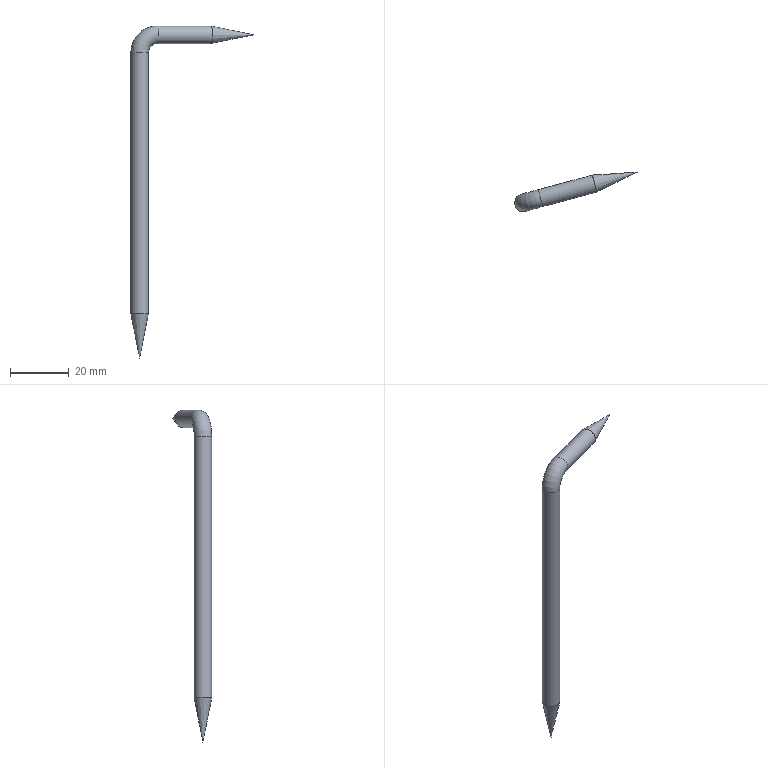Component | NX | 3 | 3 solids | 9 faces | box 41.64 x 13.41 x 113 mm | volume 3603 mm3 | plane 4 | cone 2 | cylinder 2 | torus 1 | commonest cylinder face diameters 6 x2
STEP:
#1=CARTESIAN_POINT('',(0.,0.,0.));
#2=DIRECTION('',(0.,0.,1.));
#3=DIRECTION('',(1.,0.,0.));
#4=AXIS2_PLACEMENT_3D('',#1,#2,#3);
#5=CARTESIAN_POINT('',(36.256,10.962,110.841));
#6=VERTEX_POINT('',#5);
#7=CARTESIAN_POINT('',(37.036,8.065,110.841));
#8=DIRECTION('',(0.,0.,1.));
#9=DIRECTION('',(-0.2601,0.9656,0.));
#10=AXIS2_PLACEMENT_3D('',#7,#8,#9);
#11=CIRCLE('',#10,3.);
#12=CARTESIAN_POINT('',(37.036,8.065,95.841));
#13=DIRECTION('',(0.,0.,1.));
#14=DIRECTION('',(-0.2601,0.9656,0.));
#15=AXIS2_PLACEMENT_3D('',#12,#13,#14);
#16=CONICAL_SURFACE('',#15,0.,0.1974);
#17=CARTESIAN_POINT('',(0.,15.));
#18=DIRECTION('',(1.,0.));
#19=VECTOR('',#18,1.);
#20=LINE('',#17,#19);
#21=(GEOMETRIC_REPRESENTATION_CONTEXT(2)PARAMETRIC_REPRESENTATION_CONTEXT()REPRESENTATION_CONTEXT('',''));
#22=DEFINITIONAL_REPRESENTATION('',(#20),#21);
#23=PCURVE('',#16,#22);
#24=CARTESIAN_POINT('',(39.933,8.846,110.841));
#25=DIRECTION('',(0.,0.,-1.));
#26=DIRECTION('',(0.2601,-0.9656,0.));
#27=AXIS2_PLACEMENT_3D('',#24,#25,#26);
#28=PLANE('',#27);
#29=CARTESIAN_POINT('',(-3.,3.));
#30=CARTESIAN_POINT('',(-3.,8.196));
#31=CARTESIAN_POINT('',(1.5,5.598));
#32=CARTESIAN_POINT('',(6.,3.));
#33=CARTESIAN_POINT('',(1.5,0.4019));
#34=CARTESIAN_POINT('',(-3.,-2.196));
#35=CARTESIAN_POINT('',(-3.,3.));
#36=(BOUNDED_CURVE()B_SPLINE_CURVE(2,(#29,#30,#31,#32,#33,#34,#35),.UNSPECIFIED.,.T.,.F.)B_SPLINE_CURVE_WITH_KNOTS((1,2,2,2,2,1),(-2.094,0.,2.094,4.189,6.283,8.378),.UNSPECIFIED.)CURVE()GEOMETRIC_REPRESENTATION_ITEM()RATIONAL_B_SPLINE_CURVE((1.,0.5,1.,0.5,1.,0.5,1.))REPRESENTATION_ITEM(''));
#37=(GEOMETRIC_REPRESENTATION_CONTEXT(2)PARAMETRIC_REPRESENTATION_CONTEXT()REPRESENTATION_CONTEXT('',''));
#38=DEFINITIONAL_REPRESENTATION('',(#36),#37);
#39=PCURVE('',#28,#38);
#40=SURFACE_CURVE('',#11,(#23,#39),.PCURVE_S1.);
#41=EDGE_CURVE('',#6,#6,#40,.T.);
#42=ORIENTED_EDGE('',*,*,#41,.F.);
#43=CARTESIAN_POINT('',(37.036,8.065,95.841));
#44=VERTEX_POINT('',#43);
#45=CARTESIAN_POINT('',(37.036,8.065,95.841));
#46=CARTESIAN_POINT('',(36.256,10.962,110.841));
#47=B_SPLINE_CURVE_WITH_KNOTS('',1,(#45,#46),.UNSPECIFIED.,.F.,.F.,(2,2),(-0.,15.297),.PIECEWISE_BEZIER_KNOTS.);
#48=CARTESIAN_POINT('',(0.,0.));
#49=DIRECTION('',(0.,1.));
#50=VECTOR('',#49,1.);
#51=LINE('',#48,#50);
#52=(GEOMETRIC_REPRESENTATION_CONTEXT(2)PARAMETRIC_REPRESENTATION_CONTEXT()REPRESENTATION_CONTEXT('',''));
#53=DEFINITIONAL_REPRESENTATION('',(#51),#52);
#54=PCURVE('',#16,#53);
#55=CARTESIAN_POINT('',(6.283,0.));
#56=DIRECTION('',(0.,1.));
#57=VECTOR('',#56,1.);
#58=LINE('',#55,#57);
#59=(GEOMETRIC_REPRESENTATION_CONTEXT(2)PARAMETRIC_REPRESENTATION_CONTEXT()REPRESENTATION_CONTEXT('',''));
#60=DEFINITIONAL_REPRESENTATION('',(#58),#59);
#61=PCURVE('',#16,#60);
#62=SEAM_CURVE('',#47,(#54,#61),.PCURVE_S1.);
#63=EDGE_CURVE('',#44,#6,#62,.T.);
#64=ORIENTED_EDGE('',*,*,#63,.F.);
#65=ORIENTED_EDGE('',*,*,#63,.T.);
#66=EDGE_LOOP('',(#42,#64,#65));
#67=FACE_BOUND('',#66,.T.);
#68=ADVANCED_FACE('',(#67),#16,.T.);
#69=ORIENTED_EDGE('',*,*,#41,.T.);
#70=EDGE_LOOP('',(#69));
#71=FACE_BOUND('',#70,.T.);
#72=ADVANCED_FACE('',(#71),#28,.F.);
#73=CLOSED_SHELL('',(#68,#72));
#74=MANIFOLD_SOLID_BREP('',#73);
#75=(LENGTH_UNIT()NAMED_UNIT(*)SI_UNIT(.MILLI.,.METRE.));
#76=UNCERTAINTY_MEASURE_WITH_UNIT(LENGTH_MEASURE(0.00001),#75,'','');
#77=(NAMED_UNIT(*)PLANE_ANGLE_UNIT()SI_UNIT($,.RADIAN.));
#78=(NAMED_UNIT(*)SI_UNIT($,.STERADIAN.)SOLID_ANGLE_UNIT());
#79=(GEOMETRIC_REPRESENTATION_CONTEXT(3)GLOBAL_UNCERTAINTY_ASSIGNED_CONTEXT((#76))GLOBAL_UNIT_ASSIGNED_CONTEXT((#75,#77,#78))REPRESENTATION_CONTEXT('',''));
#80=ADVANCED_BREP_SHAPE_REPRESENTATION('',(#4,#74),#79);
#81=CARTESIAN_POINT('',(0.,0.,0.));
#82=DIRECTION('',(0.,0.,1.));
#83=DIRECTION('',(1.,0.,0.));
#84=AXIS2_PLACEMENT_3D('',#81,#82,#83);
#85=CARTESIAN_POINT('',(0.,0.,0.));
#86=DIRECTION('',(0.,0.,1.));
#87=DIRECTION('',(1.,0.,0.));
#88=AXIS2_PLACEMENT_3D('',#85,#86,#87);
#89=CARTESIAN_POINT('',(0.,0.,0.));
#90=DIRECTION('',(0.,0.,1.));
#91=DIRECTION('',(1.,0.,0.));
#92=AXIS2_PLACEMENT_3D('',#89,#90,#91);
#93=(LENGTH_UNIT()NAMED_UNIT(*)SI_UNIT(.MILLI.,.METRE.));
#94=UNCERTAINTY_MEASURE_WITH_UNIT(LENGTH_MEASURE(0.00001),#93,'','');
#95=(NAMED_UNIT(*)PLANE_ANGLE_UNIT()SI_UNIT($,.RADIAN.));
#96=(NAMED_UNIT(*)SI_UNIT($,.STERADIAN.)SOLID_ANGLE_UNIT());
#97=(GEOMETRIC_REPRESENTATION_CONTEXT(3)GLOBAL_UNCERTAINTY_ASSIGNED_CONTEXT((#94))GLOBAL_UNIT_ASSIGNED_CONTEXT((#93,#95,#96))REPRESENTATION_CONTEXT('',''));
#98=SHAPE_REPRESENTATION('',(#4,#84,#88,#92),#97);
#99=ITEM_DEFINED_TRANSFORMATION('','',#4,#84);
#100=(REPRESENTATION_RELATIONSHIP('','',#80,#98)REPRESENTATION_RELATIONSHIP_WITH_TRANSFORMATION(#99)SHAPE_REPRESENTATION_RELATIONSHIP());
#101=CARTESIAN_POINT('',(42.829,9.626,208.841));
#102=VERTEX_POINT('',#101);
#103=CARTESIAN_POINT('',(42.829,9.626,205.841));
#104=DIRECTION('',(0.9656,0.2601,0.));
#105=DIRECTION('',(-0.,-0.,1.));
#106=AXIS2_PLACEMENT_3D('',#103,#104,#105);
#107=CIRCLE('',#106,3.);
#108=CARTESIAN_POINT('',(42.829,9.626,205.841));
#109=DIRECTION('',(0.9656,0.2601,0.));
#110=DIRECTION('',(-0.2601,0.9656,0.));
#111=AXIS2_PLACEMENT_3D('',#108,#109,#110);
#112=CYLINDRICAL_SURFACE('',#111,3.);
#113=CARTESIAN_POINT('',(1.571,0.));
#114=DIRECTION('',(1.,0.));
#115=VECTOR('',#114,1.);
#116=LINE('',#113,#115);
#117=(GEOMETRIC_REPRESENTATION_CONTEXT(2)PARAMETRIC_REPRESENTATION_CONTEXT()REPRESENTATION_CONTEXT('',''));
#118=DEFINITIONAL_REPRESENTATION('',(#116),#117);
#119=PCURVE('',#112,#118);
#120=CARTESIAN_POINT('',(42.829,9.626,199.841));
#121=DIRECTION('',(-0.2601,0.9656,0.));
#122=DIRECTION('',(-0.9656,-0.2601,0.));
#123=AXIS2_PLACEMENT_3D('',#120,#121,#122);
#124=TOROIDAL_SURFACE('',#123,6.,3.);
#125=CARTESIAN_POINT('',(7.854,6.283));
#126=DIRECTION('',(0.,-1.));
#127=VECTOR('',#126,1.);
#128=LINE('',#125,#127);
#129=(GEOMETRIC_REPRESENTATION_CONTEXT(2)PARAMETRIC_REPRESENTATION_CONTEXT()REPRESENTATION_CONTEXT('',''));
#130=DEFINITIONAL_REPRESENTATION('',(#128),#129);
#131=PCURVE('',#124,#130);
#132=SURFACE_CURVE('',#107,(#119,#131),.PCURVE_S1.);
#133=EDGE_CURVE('',#102,#102,#132,.T.);
#134=ORIENTED_EDGE('',*,*,#133,.T.);
#135=CARTESIAN_POINT('',(61.176,14.567,208.841));
#136=VERTEX_POINT('',#135);
#137=CARTESIAN_POINT('',(42.829,9.626,208.841));
#138=CARTESIAN_POINT('',(61.176,14.567,208.841));
#139=B_SPLINE_CURVE_WITH_KNOTS('',1,(#137,#138),.UNSPECIFIED.,.F.,.F.,(2,2),(0.,19.),.PIECEWISE_BEZIER_KNOTS.);
#140=CARTESIAN_POINT('',(7.854,0.));
#141=DIRECTION('',(0.,1.));
#142=VECTOR('',#141,1.);
#143=LINE('',#140,#142);
#144=(GEOMETRIC_REPRESENTATION_CONTEXT(2)PARAMETRIC_REPRESENTATION_CONTEXT()REPRESENTATION_CONTEXT('',''));
#145=DEFINITIONAL_REPRESENTATION('',(#143),#144);
#146=PCURVE('',#112,#145);
#147=CARTESIAN_POINT('',(1.571,0.));
#148=DIRECTION('',(0.,1.));
#149=VECTOR('',#148,1.);
#150=LINE('',#147,#149);
#151=(GEOMETRIC_REPRESENTATION_CONTEXT(2)PARAMETRIC_REPRESENTATION_CONTEXT()REPRESENTATION_CONTEXT('',''));
#152=DEFINITIONAL_REPRESENTATION('',(#150),#151);
#153=PCURVE('',#112,#152);
#154=SEAM_CURVE('',#139,(#146,#153),.PCURVE_S1.);
#155=EDGE_CURVE('',#102,#136,#154,.T.);
#156=ORIENTED_EDGE('',*,*,#155,.T.);
#157=CARTESIAN_POINT('',(61.176,14.567,205.841));
#158=DIRECTION('',(0.9656,0.2601,0.));
#159=DIRECTION('',(-0.,-0.,1.));
#160=AXIS2_PLACEMENT_3D('',#157,#158,#159);
#161=CIRCLE('',#160,3.);
#162=CARTESIAN_POINT('',(1.571,19.));
#163=DIRECTION('',(1.,0.));
#164=VECTOR('',#163,1.);
#165=LINE('',#162,#164);
#166=(GEOMETRIC_REPRESENTATION_CONTEXT(2)PARAMETRIC_REPRESENTATION_CONTEXT()REPRESENTATION_CONTEXT('',''));
#167=DEFINITIONAL_REPRESENTATION('',(#165),#166);
#168=PCURVE('',#112,#167);
#169=CARTESIAN_POINT('',(61.176,14.567,205.841));
#170=DIRECTION('',(0.9656,0.2601,0.));
#171=DIRECTION('',(-0.2601,0.9656,0.));
#172=AXIS2_PLACEMENT_3D('',#169,#170,#171);
#173=PLANE('',#172);
#174=CARTESIAN_POINT('',(0.,0.));
#175=DIRECTION('',(0.,1.));
#176=AXIS2_PLACEMENT_2D('',#174,#175);
#177=CIRCLE('',#176,3.);
#178=(GEOMETRIC_REPRESENTATION_CONTEXT(2)PARAMETRIC_REPRESENTATION_CONTEXT()REPRESENTATION_CONTEXT('',''));
#179=DEFINITIONAL_REPRESENTATION('',(#177),#178);
#180=PCURVE('',#173,#179);
#181=SURFACE_CURVE('',#161,(#168,#180),.PCURVE_S1.);
#182=EDGE_CURVE('',#136,#136,#181,.T.);
#183=ORIENTED_EDGE('',*,*,#182,.F.);
#184=ORIENTED_EDGE('',*,*,#155,.F.);
#185=EDGE_LOOP('',(#134,#156,#183,#184));
#186=FACE_BOUND('',#185,.T.);
#187=ADVANCED_FACE('',(#186),#112,.T.);
#188=CARTESIAN_POINT('',(34.139,7.285,199.841));
#189=VERTEX_POINT('',#188);
#190=CARTESIAN_POINT('',(37.036,8.065,199.841));
#191=DIRECTION('',(0.,0.,1.));
#192=DIRECTION('',(-0.9656,-0.2601,0.));
#193=AXIS2_PLACEMENT_3D('',#190,#191,#192);
#194=CIRCLE('',#193,3.);
#195=CARTESIAN_POINT('',(6.283,6.283));
#196=DIRECTION('',(0.,-1.));
#197=VECTOR('',#196,1.);
#198=LINE('',#195,#197);
#199=(GEOMETRIC_REPRESENTATION_CONTEXT(2)PARAMETRIC_REPRESENTATION_CONTEXT()REPRESENTATION_CONTEXT('',''));
#200=DEFINITIONAL_REPRESENTATION('',(#198),#199);
#201=PCURVE('',#124,#200);
#202=CARTESIAN_POINT('',(37.036,8.065,199.841));
#203=DIRECTION('',(0.,0.,-1.));
#204=DIRECTION('',(0.2601,-0.9656,0.));
#205=AXIS2_PLACEMENT_3D('',#202,#203,#204);
#206=CYLINDRICAL_SURFACE('',#205,3.);
#207=CARTESIAN_POINT('',(7.854,0.));
#208=DIRECTION('',(-1.,0.));
#209=VECTOR('',#208,1.);
#210=LINE('',#207,#209);
#211=(GEOMETRIC_REPRESENTATION_CONTEXT(2)PARAMETRIC_REPRESENTATION_CONTEXT()REPRESENTATION_CONTEXT('',''));
#212=DEFINITIONAL_REPRESENTATION('',(#210),#211);
#213=PCURVE('',#206,#212);
#214=SURFACE_CURVE('',#194,(#201,#213),.PCURVE_S1.);
#215=EDGE_CURVE('',#189,#189,#214,.T.);
#216=ORIENTED_EDGE('',*,*,#215,.T.);
#217=CARTESIAN_POINT('',(34.139,7.285,199.841));
#218=CARTESIAN_POINT('',(34.139,7.285,202.247));
#219=CARTESIAN_POINT('',(34.878,7.484,204.59));
#220=CARTESIAN_POINT('',(36.295,7.866,206.608));
#221=CARTESIAN_POINT('',(38.243,8.391,208.075));
#222=CARTESIAN_POINT('',(40.506,9.,208.841));
#223=CARTESIAN_POINT('',(42.829,9.626,208.841));
#224=(BOUNDED_CURVE()B_SPLINE_CURVE(6,(#217,#218,#219,#220,#221,#222,#223),.UNSPECIFIED.,.F.,.F.)B_SPLINE_CURVE_WITH_KNOTS((7,7),(0.,1.571),.PIECEWISE_BEZIER_KNOTS.)CURVE()GEOMETRIC_REPRESENTATION_ITEM()RATIONAL_B_SPLINE_CURVE((1.031,1.01,0.9979,0.994,0.9979,1.01,1.031))REPRESENTATION_ITEM(''));
#225=CARTESIAN_POINT('',(6.283,0.));
#226=DIRECTION('',(1.,0.));
#227=VECTOR('',#226,1.);
#228=LINE('',#225,#227);
#229=(GEOMETRIC_REPRESENTATION_CONTEXT(2)PARAMETRIC_REPRESENTATION_CONTEXT()REPRESENTATION_CONTEXT('',''));
#230=DEFINITIONAL_REPRESENTATION('',(#228),#229);
#231=PCURVE('',#124,#230);
#232=CARTESIAN_POINT('',(6.283,6.283));
#233=DIRECTION('',(1.,0.));
#234=VECTOR('',#233,1.);
#235=LINE('',#232,#234);
#236=(GEOMETRIC_REPRESENTATION_CONTEXT(2)PARAMETRIC_REPRESENTATION_CONTEXT()REPRESENTATION_CONTEXT('',''));
#237=DEFINITIONAL_REPRESENTATION('',(#235),#236);
#238=PCURVE('',#124,#237);
#239=SEAM_CURVE('',#224,(#231,#238),.PCURVE_S1.);
#240=EDGE_CURVE('',#189,#102,#239,.T.);
#241=ORIENTED_EDGE('',*,*,#240,.T.);
#242=ORIENTED_EDGE('',*,*,#133,.F.);
#243=ORIENTED_EDGE('',*,*,#240,.F.);
#244=EDGE_LOOP('',(#216,#241,#242,#243));
#245=FACE_BOUND('',#244,.T.);
#246=ADVANCED_FACE('',(#245),#124,.T.);
#247=ORIENTED_EDGE('',*,*,#215,.F.);
#248=CARTESIAN_POINT('',(34.139,7.285,110.841));
#249=VERTEX_POINT('',#248);
#250=CARTESIAN_POINT('',(34.139,7.285,199.841));
#251=CARTESIAN_POINT('',(34.139,7.285,110.841));
#252=B_SPLINE_CURVE_WITH_KNOTS('',1,(#250,#251),.UNSPECIFIED.,.F.,.F.,(2,2),(0.,89.),.PIECEWISE_BEZIER_KNOTS.);
#253=CARTESIAN_POINT('',(7.854,0.));
#254=DIRECTION('',(0.,1.));
#255=VECTOR('',#254,1.);
#256=LINE('',#253,#255);
#257=(GEOMETRIC_REPRESENTATION_CONTEXT(2)PARAMETRIC_REPRESENTATION_CONTEXT()REPRESENTATION_CONTEXT('',''));
#258=DEFINITIONAL_REPRESENTATION('',(#256),#257);
#259=PCURVE('',#206,#258);
#260=CARTESIAN_POINT('',(1.571,0.));
#261=DIRECTION('',(0.,1.));
#262=VECTOR('',#261,1.);
#263=LINE('',#260,#262);
#264=(GEOMETRIC_REPRESENTATION_CONTEXT(2)PARAMETRIC_REPRESENTATION_CONTEXT()REPRESENTATION_CONTEXT('',''));
#265=DEFINITIONAL_REPRESENTATION('',(#263),#264);
#266=PCURVE('',#206,#265);
#267=SEAM_CURVE('',#252,(#259,#266),.PCURVE_S1.);
#268=EDGE_CURVE('',#189,#249,#267,.T.);
#269=ORIENTED_EDGE('',*,*,#268,.T.);
#270=CARTESIAN_POINT('',(37.036,8.065,110.841));
#271=DIRECTION('',(0.,0.,1.));
#272=DIRECTION('',(-0.9656,-0.2601,0.));
#273=AXIS2_PLACEMENT_3D('',#270,#271,#272);
#274=CIRCLE('',#273,3.);
#275=CARTESIAN_POINT('',(7.854,89.));
#276=DIRECTION('',(-1.,0.));
#277=VECTOR('',#276,1.);
#278=LINE('',#275,#277);
#279=(GEOMETRIC_REPRESENTATION_CONTEXT(2)PARAMETRIC_REPRESENTATION_CONTEXT()REPRESENTATION_CONTEXT('',''));
#280=DEFINITIONAL_REPRESENTATION('',(#278),#279);
#281=PCURVE('',#206,#280);
#282=CARTESIAN_POINT('',(37.036,8.065,110.841));
#283=DIRECTION('',(0.,0.,1.));
#284=DIRECTION('',(-0.2601,0.9656,0.));
#285=AXIS2_PLACEMENT_3D('',#282,#283,#284);
#286=PLANE('',#285);
#287=CARTESIAN_POINT('',(0.,0.));
#288=DIRECTION('',(0.,1.));
#289=AXIS2_PLACEMENT_2D('',#287,#288);
#290=CIRCLE('',#289,3.);
#291=(GEOMETRIC_REPRESENTATION_CONTEXT(2)PARAMETRIC_REPRESENTATION_CONTEXT()REPRESENTATION_CONTEXT('',''));
#292=DEFINITIONAL_REPRESENTATION('',(#290),#291);
#293=PCURVE('',#286,#292);
#294=SURFACE_CURVE('',#274,(#281,#293),.PCURVE_S1.);
#295=EDGE_CURVE('',#249,#249,#294,.T.);
#296=ORIENTED_EDGE('',*,*,#295,.T.);
#297=ORIENTED_EDGE('',*,*,#268,.F.);
#298=EDGE_LOOP('',(#247,#269,#296,#297));
#299=FACE_BOUND('',#298,.T.);
#300=ADVANCED_FACE('',(#299),#206,.T.);
#301=ORIENTED_EDGE('',*,*,#182,.T.);
#302=EDGE_LOOP('',(#301));
#303=FACE_BOUND('',#302,.T.);
#304=ADVANCED_FACE('',(#303),#173,.T.);
#305=ORIENTED_EDGE('',*,*,#295,.F.);
#306=EDGE_LOOP('',(#305));
#307=FACE_BOUND('',#306,.T.);
#308=ADVANCED_FACE('',(#307),#286,.F.);
#309=CLOSED_SHELL('',(#187,#246,#300,#304,#308));
#310=MANIFOLD_SOLID_BREP('',#309);
#311=(LENGTH_UNIT()NAMED_UNIT(*)SI_UNIT(.MILLI.,.METRE.));
#312=UNCERTAINTY_MEASURE_WITH_UNIT(LENGTH_MEASURE(0.00001),#311,'','');
#313=(NAMED_UNIT(*)PLANE_ANGLE_UNIT()SI_UNIT($,.RADIAN.));
#314=(NAMED_UNIT(*)SI_UNIT($,.STERADIAN.)SOLID_ANGLE_UNIT());
#315=(GEOMETRIC_REPRESENTATION_CONTEXT(3)GLOBAL_UNCERTAINTY_ASSIGNED_CONTEXT((#312))GLOBAL_UNIT_ASSIGNED_CONTEXT((#311,#313,#314))REPRESENTATION_CONTEXT('',''));
#316=ADVANCED_BREP_SHAPE_REPRESENTATION('',(#4,#310),#315);
#317=ITEM_DEFINED_TRANSFORMATION('','',#4,#88);
#318=(REPRESENTATION_RELATIONSHIP('','',#316,#98)REPRESENTATION_RELATIONSHIP_WITH_TRANSFORMATION(#317)SHAPE_REPRESENTATION_RELATIONSHIP());
#319=CARTESIAN_POINT('',(60.395,17.464,205.841));
#320=VERTEX_POINT('',#319);
#321=CARTESIAN_POINT('',(61.956,11.67,205.841));
#322=VERTEX_POINT('',#321);
#323=CARTESIAN_POINT('',(61.176,14.567,205.841));
#324=DIRECTION('',(0.9656,0.2601,0.));
#325=DIRECTION('',(-0.2601,0.9656,0.));
#326=AXIS2_PLACEMENT_3D('',#323,#324,#325);
#327=CIRCLE('',#326,3.);
#328=CARTESIAN_POINT('',(75.677,18.473,205.841));
#329=DIRECTION('',(-0.9656,-0.2601,0.));
#330=DIRECTION('',(0.2601,-0.9656,0.));
#331=AXIS2_PLACEMENT_3D('',#328,#329,#330);
#332=CONICAL_SURFACE('',#331,0.,0.1972);
#333=CARTESIAN_POINT('',(3.142,15.019));
#334=DIRECTION('',(-1.,0.));
#335=VECTOR('',#334,1.);
#336=LINE('',#333,#335);
#337=(GEOMETRIC_REPRESENTATION_CONTEXT(2)PARAMETRIC_REPRESENTATION_CONTEXT()REPRESENTATION_CONTEXT('',''));
#338=DEFINITIONAL_REPRESENTATION('',(#336),#337);
#339=PCURVE('',#332,#338);
#340=CARTESIAN_POINT('',(61.176,14.567,208.841));
#341=DIRECTION('',(-0.9656,-0.2601,0.));
#342=DIRECTION('',(0.2601,-0.9656,0.));
#343=AXIS2_PLACEMENT_3D('',#340,#341,#342);
#344=PLANE('',#343);
#345=CARTESIAN_POINT('',(-3.,-3.));
#346=CARTESIAN_POINT('',(-3.,2.196));
#347=CARTESIAN_POINT('',(1.5,-0.4019));
#348=CARTESIAN_POINT('',(6.,-3.));
#349=CARTESIAN_POINT('',(1.5,-5.598));
#350=CARTESIAN_POINT('',(-3.,-8.196));
#351=CARTESIAN_POINT('',(-3.,-3.));
#352=(BOUNDED_CURVE()B_SPLINE_CURVE(2,(#345,#346,#347,#348,#349,#350,#351),.UNSPECIFIED.,.T.,.F.)B_SPLINE_CURVE_WITH_KNOTS((1,2,2,2,2,1),(-2.094,0.,2.094,4.189,6.283,8.378),.UNSPECIFIED.)CURVE()GEOMETRIC_REPRESENTATION_ITEM()RATIONAL_B_SPLINE_CURVE((1.,0.5,1.,0.5,1.,0.5,1.))REPRESENTATION_ITEM(''));
#353=(GEOMETRIC_REPRESENTATION_CONTEXT(2)PARAMETRIC_REPRESENTATION_CONTEXT()REPRESENTATION_CONTEXT('',''));
#354=DEFINITIONAL_REPRESENTATION('',(#352),#353);
#355=PCURVE('',#344,#354);
#356=SURFACE_CURVE('',#327,(#339,#355),.PCURVE_S1.);
#357=EDGE_CURVE('',#320,#322,#356,.T.);
#358=ORIENTED_EDGE('',*,*,#357,.T.);
#359=CARTESIAN_POINT('',(75.677,18.473,205.841));
#360=VERTEX_POINT('',#359);
#361=CARTESIAN_POINT('',(75.677,18.473,205.841));
#362=CARTESIAN_POINT('',(61.956,11.67,205.841));
#363=B_SPLINE_CURVE_WITH_KNOTS('',1,(#361,#362),.UNSPECIFIED.,.F.,.F.,(2,2),(0.,15.315),.PIECEWISE_BEZIER_KNOTS.);
#364=CARTESIAN_POINT('',(0.,0.));
#365=DIRECTION('',(0.,1.));
#366=VECTOR('',#365,1.);
#367=LINE('',#364,#366);
#368=(GEOMETRIC_REPRESENTATION_CONTEXT(2)PARAMETRIC_REPRESENTATION_CONTEXT()REPRESENTATION_CONTEXT('',''));
#369=DEFINITIONAL_REPRESENTATION('',(#367),#368);
#370=PCURVE('',#332,#369);
#371=CARTESIAN_POINT('',(6.283,0.));
#372=DIRECTION('',(0.,1.));
#373=VECTOR('',#372,1.);
#374=LINE('',#371,#373);
#375=(GEOMETRIC_REPRESENTATION_CONTEXT(2)PARAMETRIC_REPRESENTATION_CONTEXT()REPRESENTATION_CONTEXT('',''));
#376=DEFINITIONAL_REPRESENTATION('',(#374),#375);
#377=PCURVE('',#332,#376);
#378=SEAM_CURVE('',#363,(#370,#377),.PCURVE_S1.);
#379=EDGE_CURVE('',#360,#322,#378,.T.);
#380=ORIENTED_EDGE('',*,*,#379,.F.);
#381=ORIENTED_EDGE('',*,*,#379,.T.);
#382=CARTESIAN_POINT('',(61.176,14.567,205.841));
#383=DIRECTION('',(0.9656,0.2601,0.));
#384=DIRECTION('',(-0.2601,0.9656,0.));
#385=AXIS2_PLACEMENT_3D('',#382,#383,#384);
#386=CIRCLE('',#385,3.);
#387=CARTESIAN_POINT('',(9.425,15.019));
#388=DIRECTION('',(-1.,0.));
#389=VECTOR('',#388,1.);
#390=LINE('',#387,#389);
#391=(GEOMETRIC_REPRESENTATION_CONTEXT(2)PARAMETRIC_REPRESENTATION_CONTEXT()REPRESENTATION_CONTEXT('',''));
#392=DEFINITIONAL_REPRESENTATION('',(#390),#391);
#393=PCURVE('',#332,#392);
#394=CARTESIAN_POINT('',(-3.,-3.));
#395=CARTESIAN_POINT('',(-3.,2.196));
#396=CARTESIAN_POINT('',(1.5,-0.4019));
#397=CARTESIAN_POINT('',(6.,-3.));
#398=CARTESIAN_POINT('',(1.5,-5.598));
#399=CARTESIAN_POINT('',(-3.,-8.196));
#400=CARTESIAN_POINT('',(-3.,-3.));
#401=(BOUNDED_CURVE()B_SPLINE_CURVE(2,(#394,#395,#396,#397,#398,#399,#400),.UNSPECIFIED.,.T.,.F.)B_SPLINE_CURVE_WITH_KNOTS((1,2,2,2,2,1),(-2.094,0.,2.094,4.189,6.283,8.378),.UNSPECIFIED.)CURVE()GEOMETRIC_REPRESENTATION_ITEM()RATIONAL_B_SPLINE_CURVE((1.,0.5,1.,0.5,1.,0.5,1.))REPRESENTATION_ITEM(''));
#402=(GEOMETRIC_REPRESENTATION_CONTEXT(2)PARAMETRIC_REPRESENTATION_CONTEXT()REPRESENTATION_CONTEXT('',''));
#403=DEFINITIONAL_REPRESENTATION('',(#401),#402);
#404=PCURVE('',#344,#403);
#405=SURFACE_CURVE('',#386,(#393,#404),.PCURVE_S1.);
#406=EDGE_CURVE('',#322,#320,#405,.T.);
#407=ORIENTED_EDGE('',*,*,#406,.T.);
#408=EDGE_LOOP('',(#358,#380,#381,#407));
#409=FACE_BOUND('',#408,.T.);
#410=ADVANCED_FACE('',(#409),#332,.T.);
#411=ORIENTED_EDGE('',*,*,#357,.F.);
#412=ORIENTED_EDGE('',*,*,#406,.F.);
#413=EDGE_LOOP('',(#411,#412));
#414=FACE_BOUND('',#413,.T.);
#415=ADVANCED_FACE('',(#414),#344,.T.);
#416=CLOSED_SHELL('',(#410,#415));
#417=MANIFOLD_SOLID_BREP('',#416);
#418=(LENGTH_UNIT()NAMED_UNIT(*)SI_UNIT(.MILLI.,.METRE.));
#419=UNCERTAINTY_MEASURE_WITH_UNIT(LENGTH_MEASURE(0.000005),#418,'','');
#420=(NAMED_UNIT(*)PLANE_ANGLE_UNIT()SI_UNIT($,.RADIAN.));
#421=(NAMED_UNIT(*)SI_UNIT($,.STERADIAN.)SOLID_ANGLE_UNIT());
#422=(GEOMETRIC_REPRESENTATION_CONTEXT(3)GLOBAL_UNCERTAINTY_ASSIGNED_CONTEXT((#419))GLOBAL_UNIT_ASSIGNED_CONTEXT((#418,#420,#421))REPRESENTATION_CONTEXT('',''));
#423=ADVANCED_BREP_SHAPE_REPRESENTATION('',(#4,#417),#422);
#424=ITEM_DEFINED_TRANSFORMATION('','',#4,#92);
#425=(REPRESENTATION_RELATIONSHIP('','',#423,#98)REPRESENTATION_RELATIONSHIP_WITH_TRANSFORMATION(#424)SHAPE_REPRESENTATION_RELATIONSHIP());